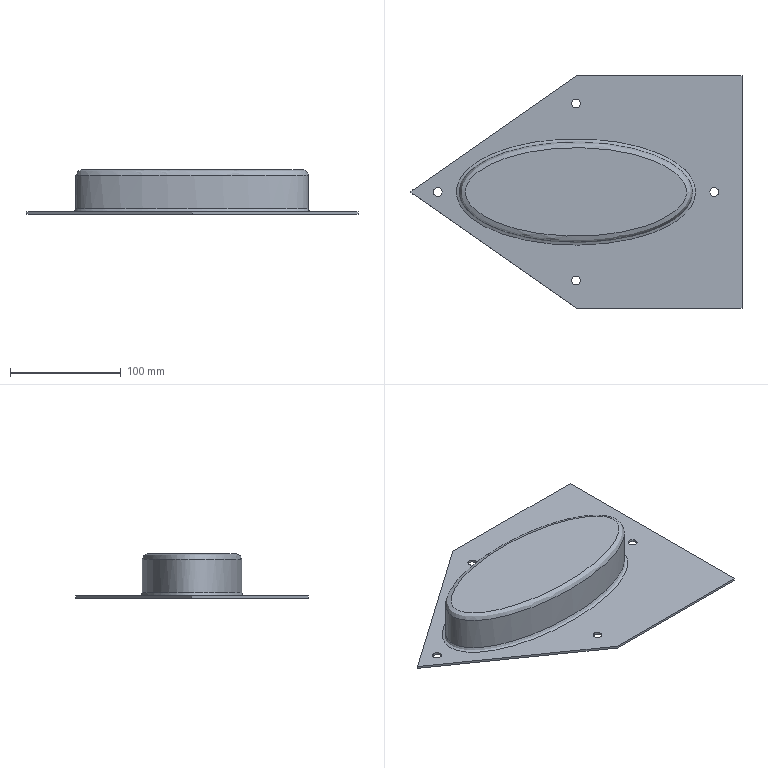Component | NX | DRAWN_PART | 1 solid | 19 faces | volume 124050 mm3 | plane 9 | spline 5 | cylinder 4 | other 1 | commonest cylinder face diameters 8.06 x4